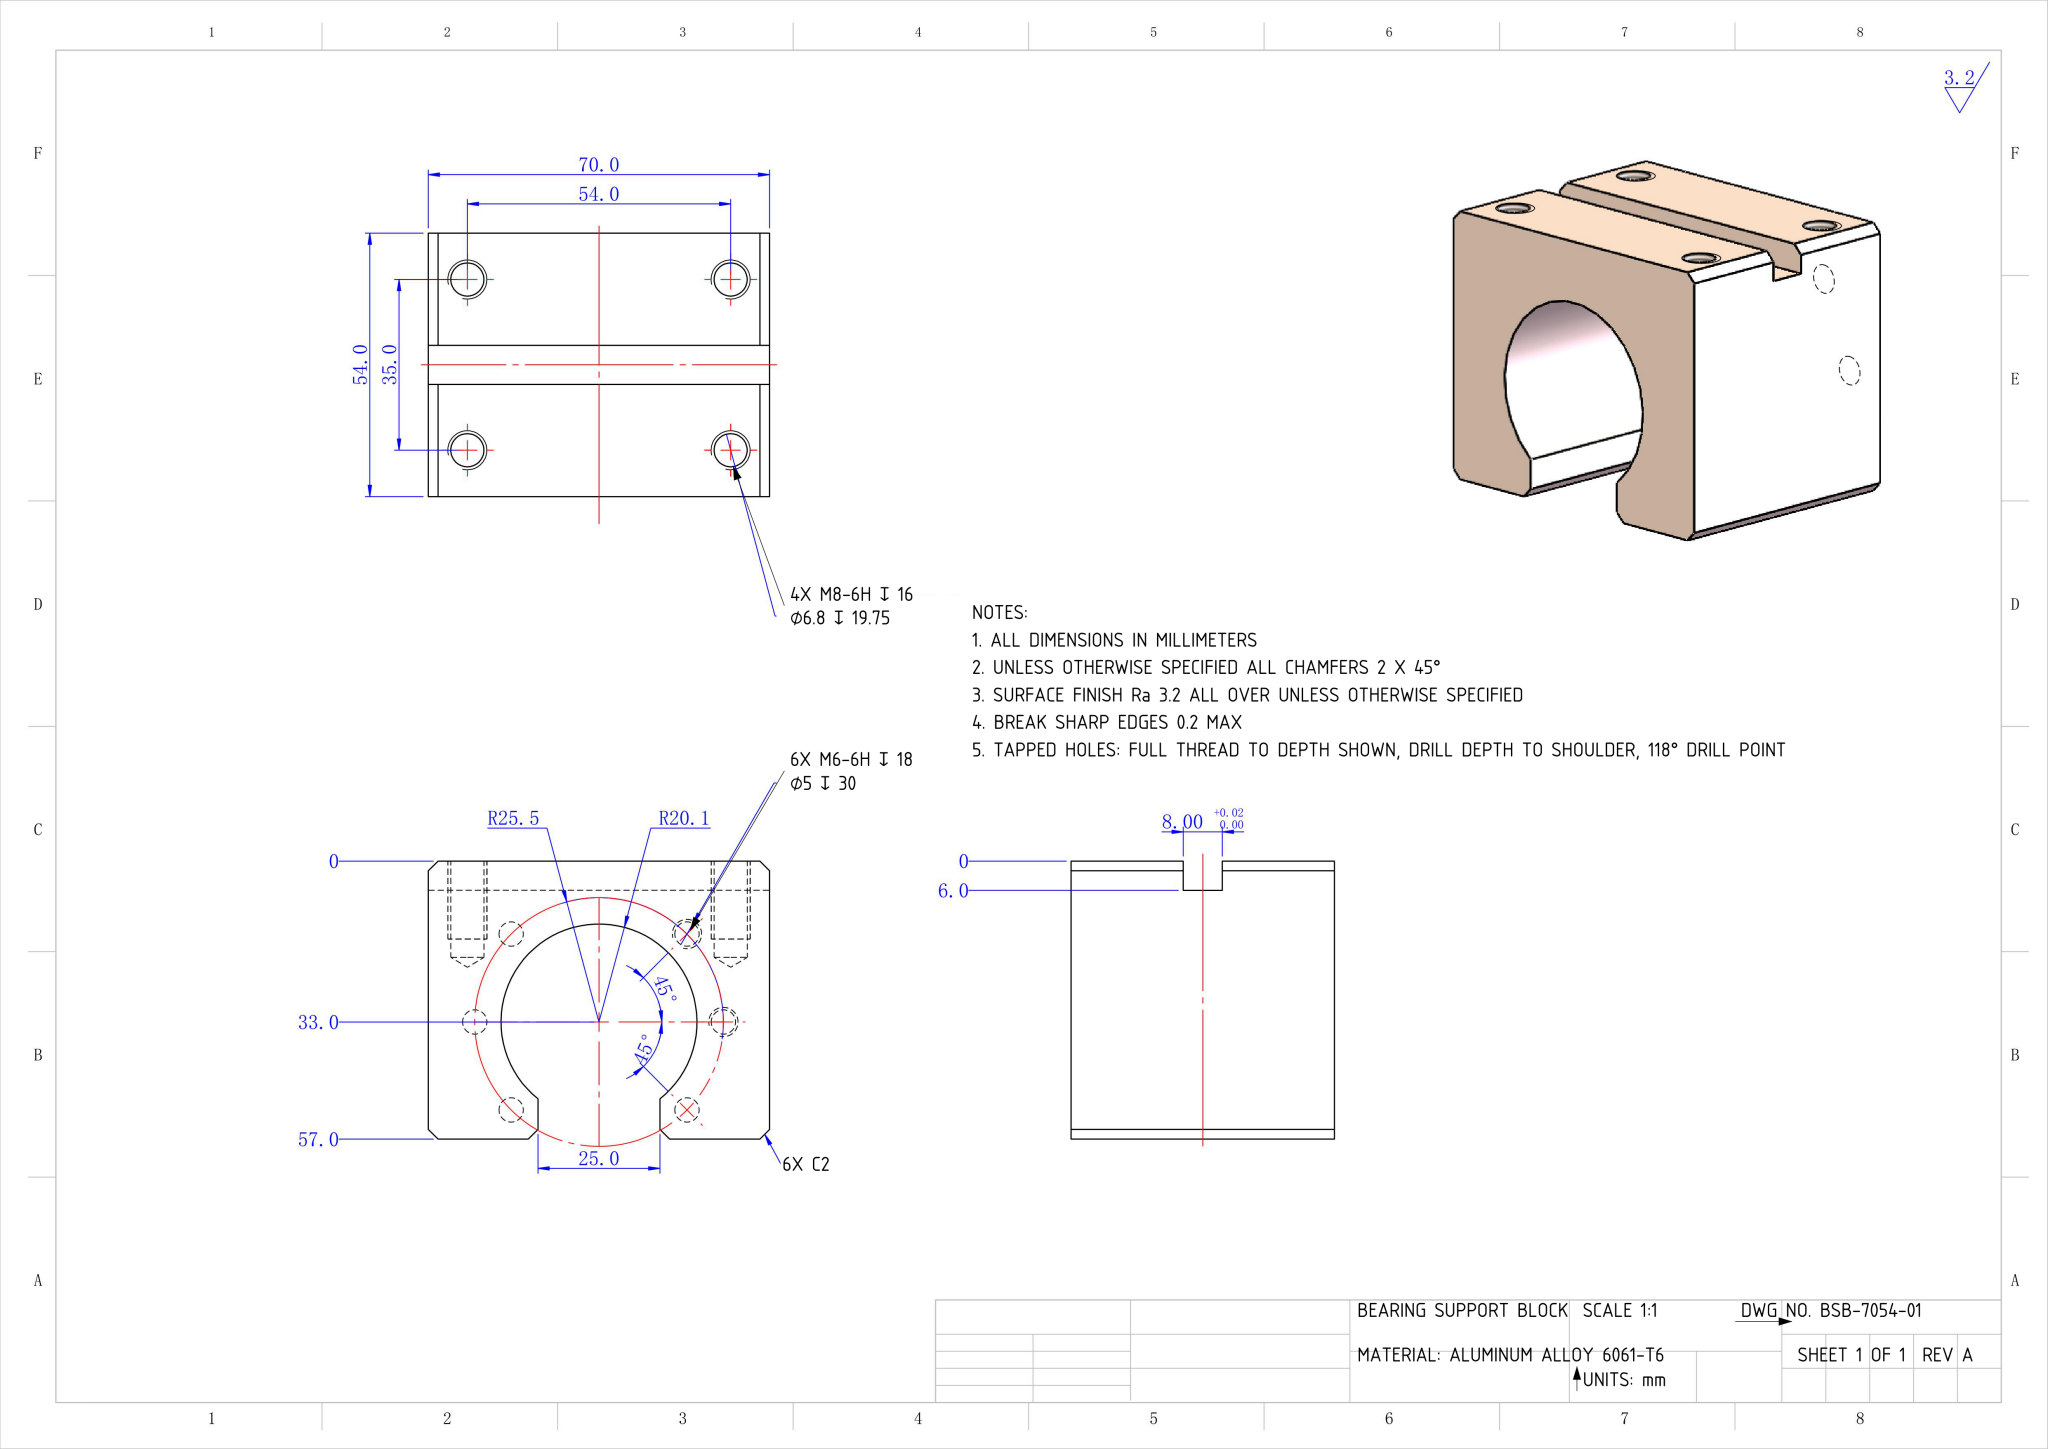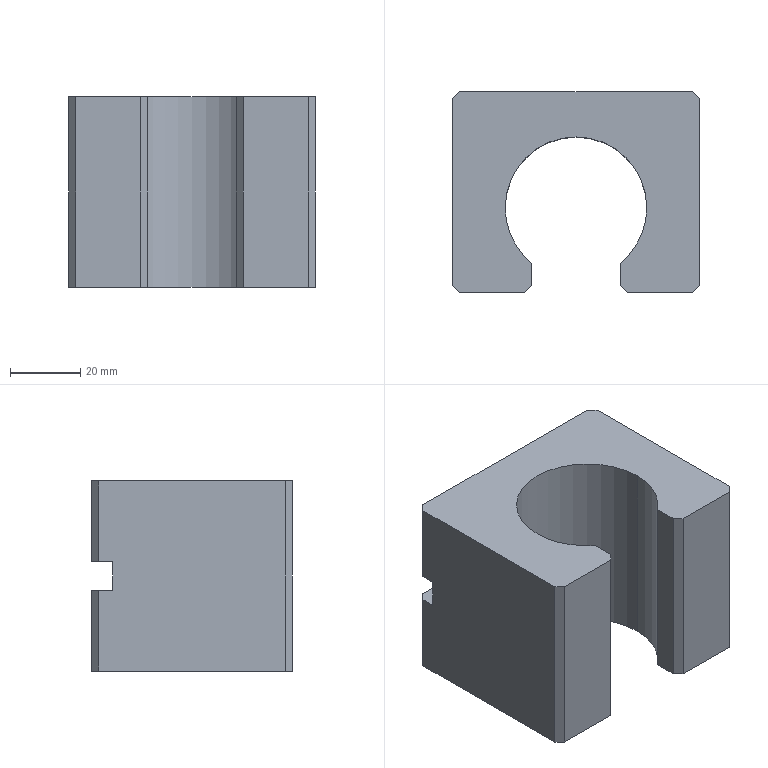Part | NX | mm | 1 solid | 64 faces | box 70 x 57 x 54 mm | volume 129251 mm3 | cylinder 23 | plane 21 | cone 20 | commonest cylinder face diameters 5 x12 6.8 x8 40.2 x3